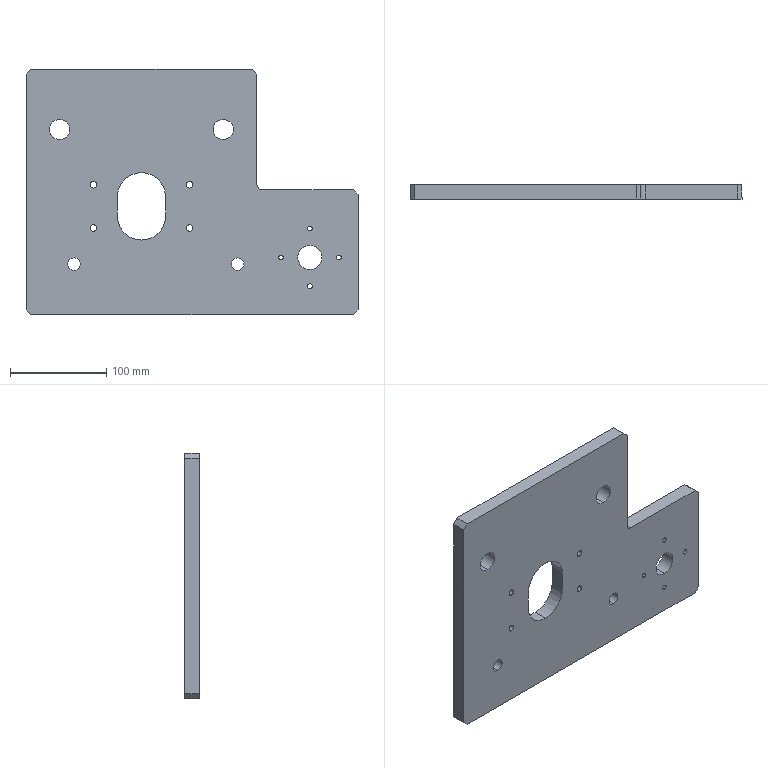Component | SolidWorks | -TractorTopPlate-1 | 1 solid | 45 faces | volume 1052348 mm3 | cylinder 30 | plane 15 | commonest cylinder face diameters 6.8 x8 5 x8 13 x4 21 x4 50 x3 25 x2 10 x1